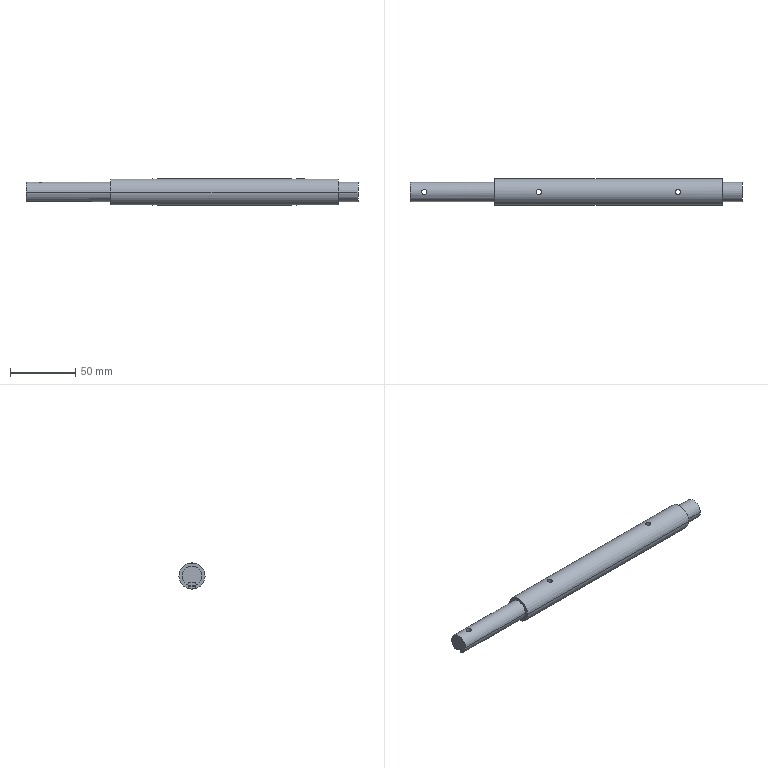Component | SolidWorks | 03-1 | 1 solid | 28 faces | box 255 x 20 x 20 mm | volume 67301 mm3 | plane 16 | cylinder 12 | commonest cylinder face diameters 4 x6 15 x4 20 x2
build123d program:
from build123d import *

# Parameters (mm, degrees)
SKETCH1_R            = 10
EXTRUDE1_DEPTH       = 95
SKETCH2_R            = 2
CUT_EXTRUDE1_DEPTH   = 10
SKETCH3_R            = 10
SKETCH3_R_2          = 7.5
EXTRUDE2_DEPTH       = 15
SKETCH4_R            = 7.5
EXTRUDE3_DEPTH       = 65
SKETCH5_W            = 5
SKETCH5_H            = 5
EXTRUDE4_DEPTH       = 50
SKETCH6_W            = 5
SKETCH6_H            = 5
EXTRUDE5_DEPTH       = 30
SKETCH7_W            = 5
SKETCH7_H            = 5
EXTRUDE6_DEPTH       = 30
SKETCH1_2_R          = 2
CUT_EXTRUDE1_2_DEPTH = 18


with BuildPart() as part:
    # Sketch1 → Extrude1 (new, symmetric)
    with BuildSketch(Plane(origin=(0, 0, 0), x_dir=(0, 0, -1), z_dir=(1, 0, 0))):
        Circle(SKETCH1_R)
    extrude(amount=EXTRUDE1_DEPTH, both=True)

    # Sketch2 → Cut-Extrude1 (cut, symmetric)
    with BuildSketch(Plane(origin=(0, 0, 0), x_dir=(1, 0, 0), z_dir=(0, 1, 0))):
        with Locations(Location((46, 0, 0), (0, 0, 270))):
            Circle(SKETCH2_R)
        with Locations(Location((-61, 0, 0), (0, 0, 270))):
            Circle(SKETCH2_R)
    extrude(amount=CUT_EXTRUDE1_DEPTH, both=True, mode=Mode.SUBTRACT)

    # Sketch3 → Extrude2 (cut)
    with BuildSketch(Plane(origin=(95, 0, 0), x_dir=(0, 0, -1), z_dir=(1, 0, 0))):
        Circle(SKETCH3_R)
        Circle(SKETCH3_R_2, mode=Mode.SUBTRACT)
    extrude(amount=-EXTRUDE2_DEPTH, mode=Mode.SUBTRACT)

    # Sketch4 → Extrude3 (add)
    with BuildSketch(Plane.ZY.offset(95)):
        with Locations(Location((0, 0, 0), (0, 0, 180))):
            Circle(SKETCH4_R)
    extrude(amount=EXTRUDE3_DEPTH)

    # Sketch5 → Extrude4 (cut)
    with BuildSketch(Plane.ZY.offset(160)):
        with Locations((0, 7.5)):
            Rectangle(SKETCH5_W, SKETCH5_H)
    extrude(amount=-EXTRUDE4_DEPTH, mode=Mode.SUBTRACT)

    # Sketch6 → Extrude5 (cut)
    with BuildSketch(Plane.ZY.offset(95)):
        with Locations((0, 10.5)):
            Rectangle(SKETCH6_W, SKETCH6_H)
    extrude(amount=-EXTRUDE5_DEPTH, mode=Mode.SUBTRACT)

    # Sketch7 → Extrude6 (cut)
    with BuildSketch(Plane(origin=(80, 0, 0), x_dir=(0, 0, -1), z_dir=(1, 0, 0))):
        with Locations((0, 10.5)):
            Rectangle(SKETCH7_W, SKETCH7_H)
    extrude(amount=-EXTRUDE6_DEPTH, mode=Mode.SUBTRACT)

    # Sketch1_2 → Cut-Extrude1_2 (cut)
    with BuildSketch(Plane(origin=(0, 5, 0), x_dir=(1, 0, 0), z_dir=(0, 1, 0))):
        with Locations(Location((-149, 0, 0), (0, 0, 270))):
            Circle(SKETCH1_2_R)
    extrude(amount=-CUT_EXTRUDE1_2_DEPTH, mode=Mode.SUBTRACT)


solid = part.part

# Placed as in the assembly
solid = solid.moved(Location((15.5, -32.5, 30), (-90, 0, 0)))